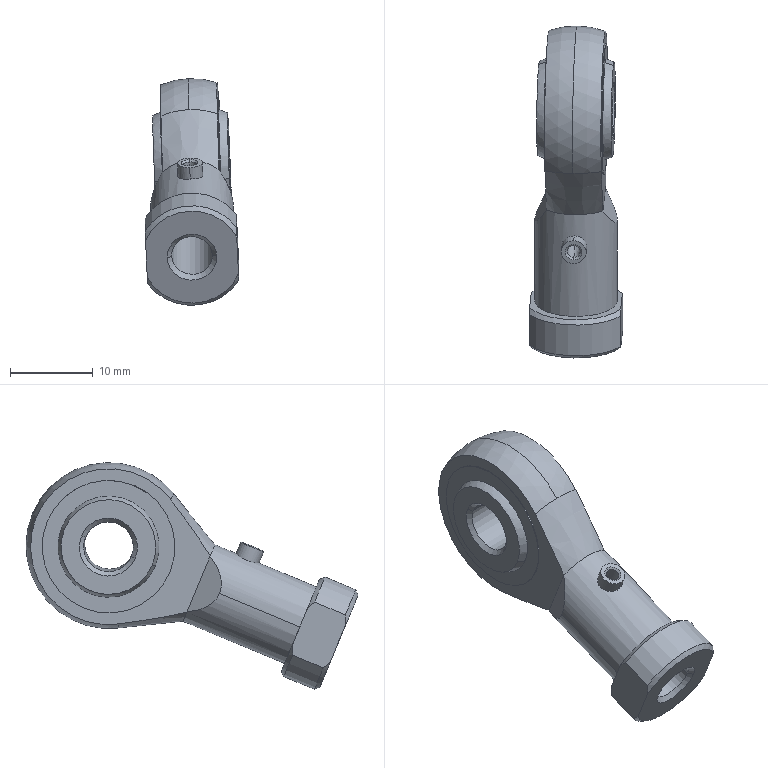Component | SolidWorks | F-M6X100U-1 | 1 solid | 53 faces | volume 3636 mm3 | cone 17 | cylinder 16 | plane 14 | spline 4 | sphere 2 | commonest cylinder face diameters 16 x4 4.917 x2 6 x2 3 x2 1.567 x2 10 x2 13 x2